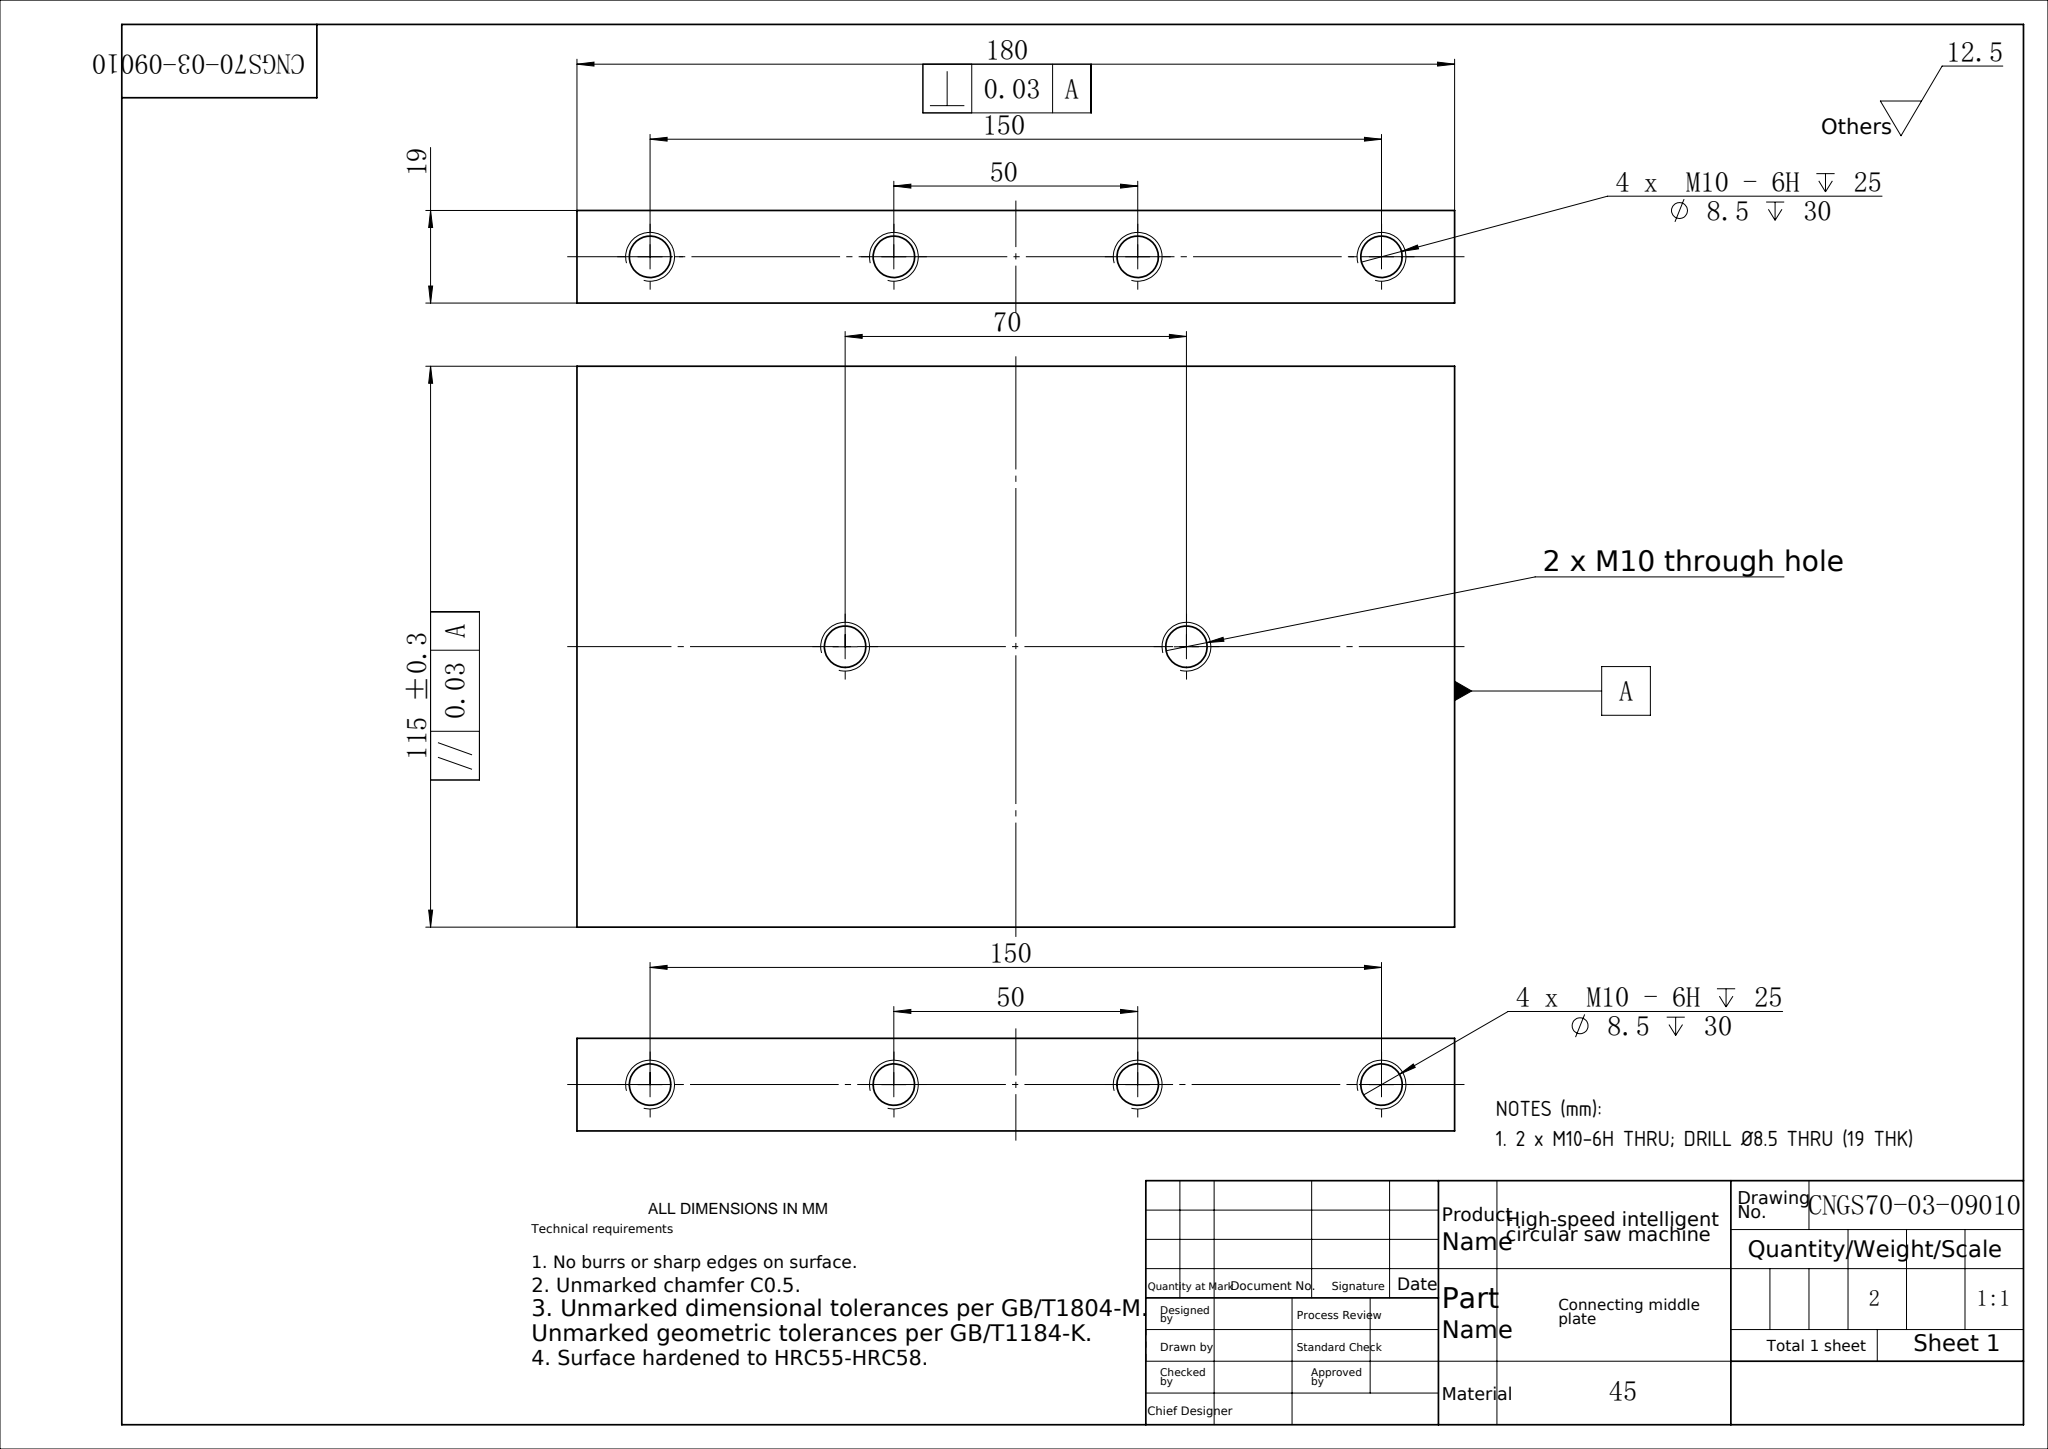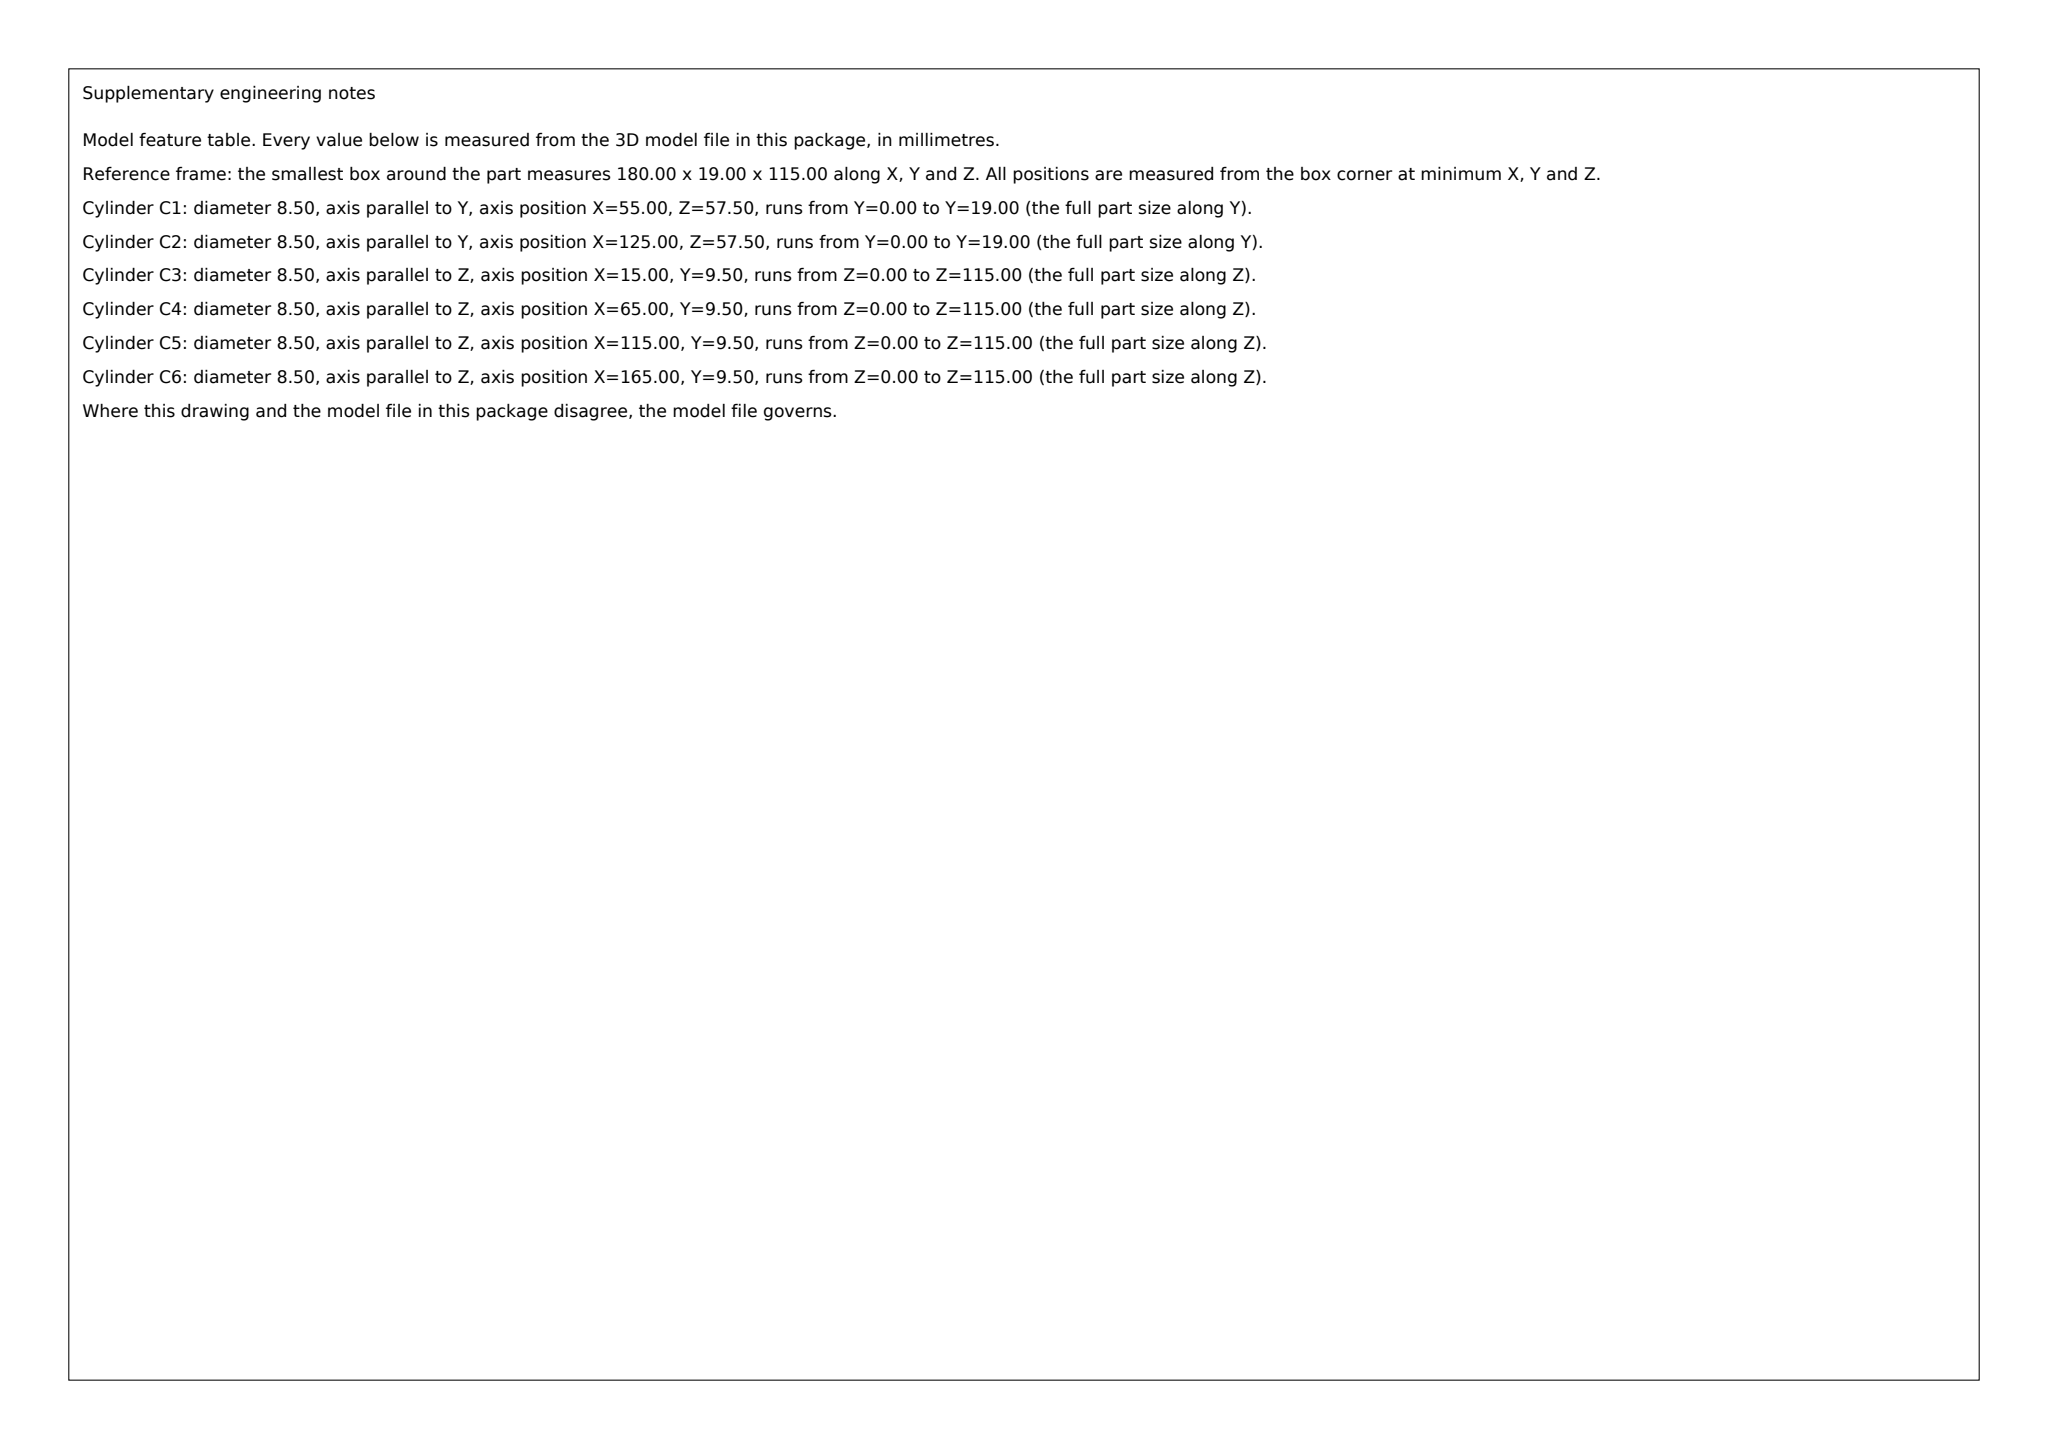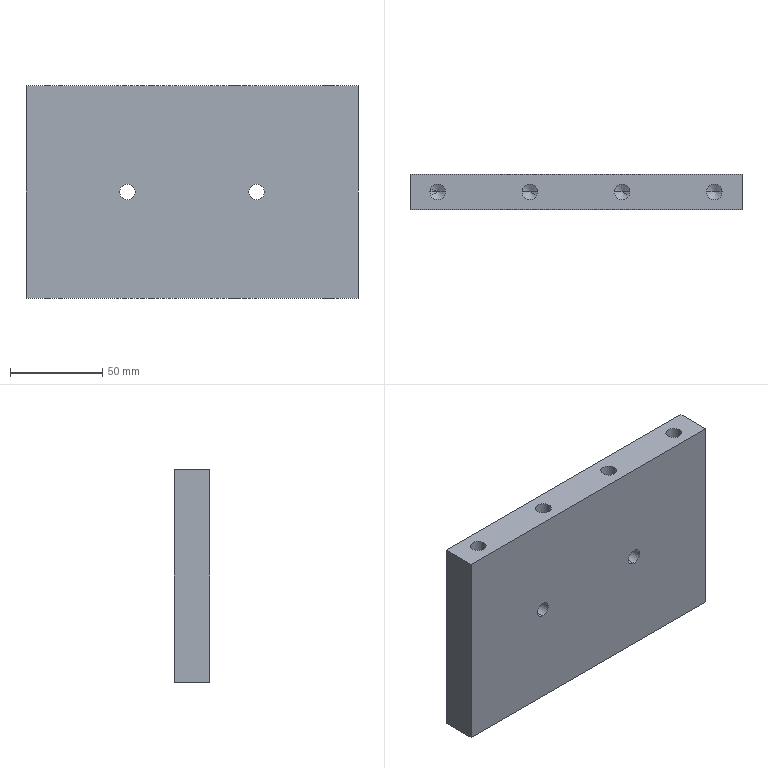Part | SolidWorks | mm | material 45 | 1 solid | 42 faces | box 180 x 19 x 115 mm | volume 377138 mm3 | cylinder 20 | cone 16 | plane 6 | commonest cylinder face diameters 8.5 x20
Drawing notes:
2 x M10-6H THRU; DRILL Ø8.5 THRU (19 THK) | from the solid: cylinders dia 8.5 axis y at (55,57.5) and (125,57.5), length 19.0 = full Y thickness (planes y=0, y=19)
build123d program:
from build123d import *

# Parameters (mm, degrees)
SKETCH1_W              = 180
SKETCH1_H              = 19
BOSS_EXTRUDE1_DEPTH    = 115
M10_TAPPED_HOLE1_D     = 8.5
M10_TAPPED_HOLE1_DEPTH = 30
M10_TAPPED_HOLE1_TIP   = 2.554
M10_TAPPED_HOLE2_D     = 8.5
M10_TAPPED_HOLE2_DEPTH = 30
M10_TAPPED_HOLE2_TIP   = 2.554
SKETCH6_R              = 3.5
CUT_EXTRUDE1_DEPTH     = 30
M10_TAPPED_HOLE3_D     = 8.5


with BuildPart() as part:
    # Sketch1 → Boss-Extrude1 (new body)
    with BuildSketch(Plane.XY):
        Rectangle(SKETCH1_W, SKETCH1_H)
    extrude(amount=BOSS_EXTRUDE1_DEPTH)

    # M10 Tapped Hole1
    with Locations(Plane.XY.offset(115)):
        with Locations((-25, 0), (25, 0), (-75, 0), (75, 0)):
            Hole(M10_TAPPED_HOLE1_D / 2, depth=M10_TAPPED_HOLE1_DEPTH)
            with Locations((0, 0, -(M10_TAPPED_HOLE1_DEPTH + M10_TAPPED_HOLE1_TIP / 2))):  # 118° drill point
                Cone(0, M10_TAPPED_HOLE1_D / 2, M10_TAPPED_HOLE1_TIP, mode=Mode.SUBTRACT)

    # M10 Tapped Hole2
    with Locations(Plane(origin=(0, 0, 0), x_dir=(-1, 0, 0), z_dir=(0, 0, -1))):
        with Locations((-25, 0), (25, 0), (75, 0), (-75, 0)):
            Hole(M10_TAPPED_HOLE2_D / 2, depth=M10_TAPPED_HOLE2_DEPTH)
            with Locations((0, 0, -(M10_TAPPED_HOLE2_DEPTH + M10_TAPPED_HOLE2_TIP / 2))):  # 118° drill point
                Cone(0, M10_TAPPED_HOLE2_D / 2, M10_TAPPED_HOLE2_TIP, mode=Mode.SUBTRACT)

    # Sketch6 → Cut-Extrude1 (cut)
    with BuildSketch(Plane(origin=(0, 9.5, 0), x_dir=(1, 0, 0), z_dir=(0, 1, 0))):
        with Locations(Location((-35, -57.5, 0), (0, 0, 270))):
            Circle(SKETCH6_R)
        with Locations(Location((35, -57.5, 0), (0, 0, 270))):
            Circle(SKETCH6_R)
    extrude(amount=-CUT_EXTRUDE1_DEPTH, mode=Mode.SUBTRACT)

    # M10 Tapped Hole3 (through all)
    with Locations(Plane(origin=(0, 9.5, 0), x_dir=(1, 0, 0), z_dir=(0, 1, 0))):
        with Locations((35, -57.5), (-35, -57.5)):
            Hole(M10_TAPPED_HOLE3_D / 2)


solid = part.part